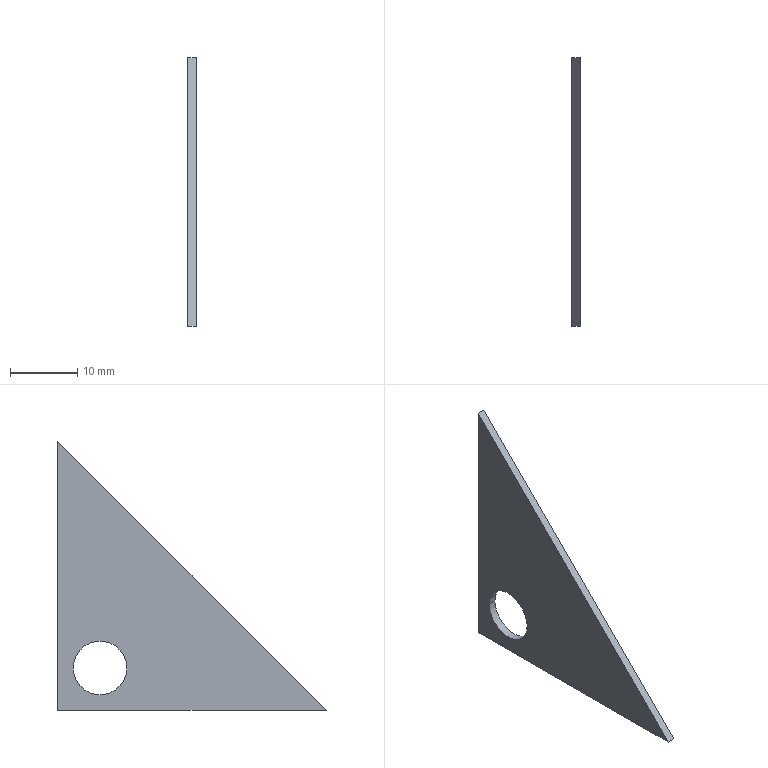Component | SolidWorks | CabinetWelding-1_Triangle-2 | 1 solid | 7 faces | volume 900 mm3 | plane 5 | cylinder 2 | commonest cylinder face diameters 8 x2